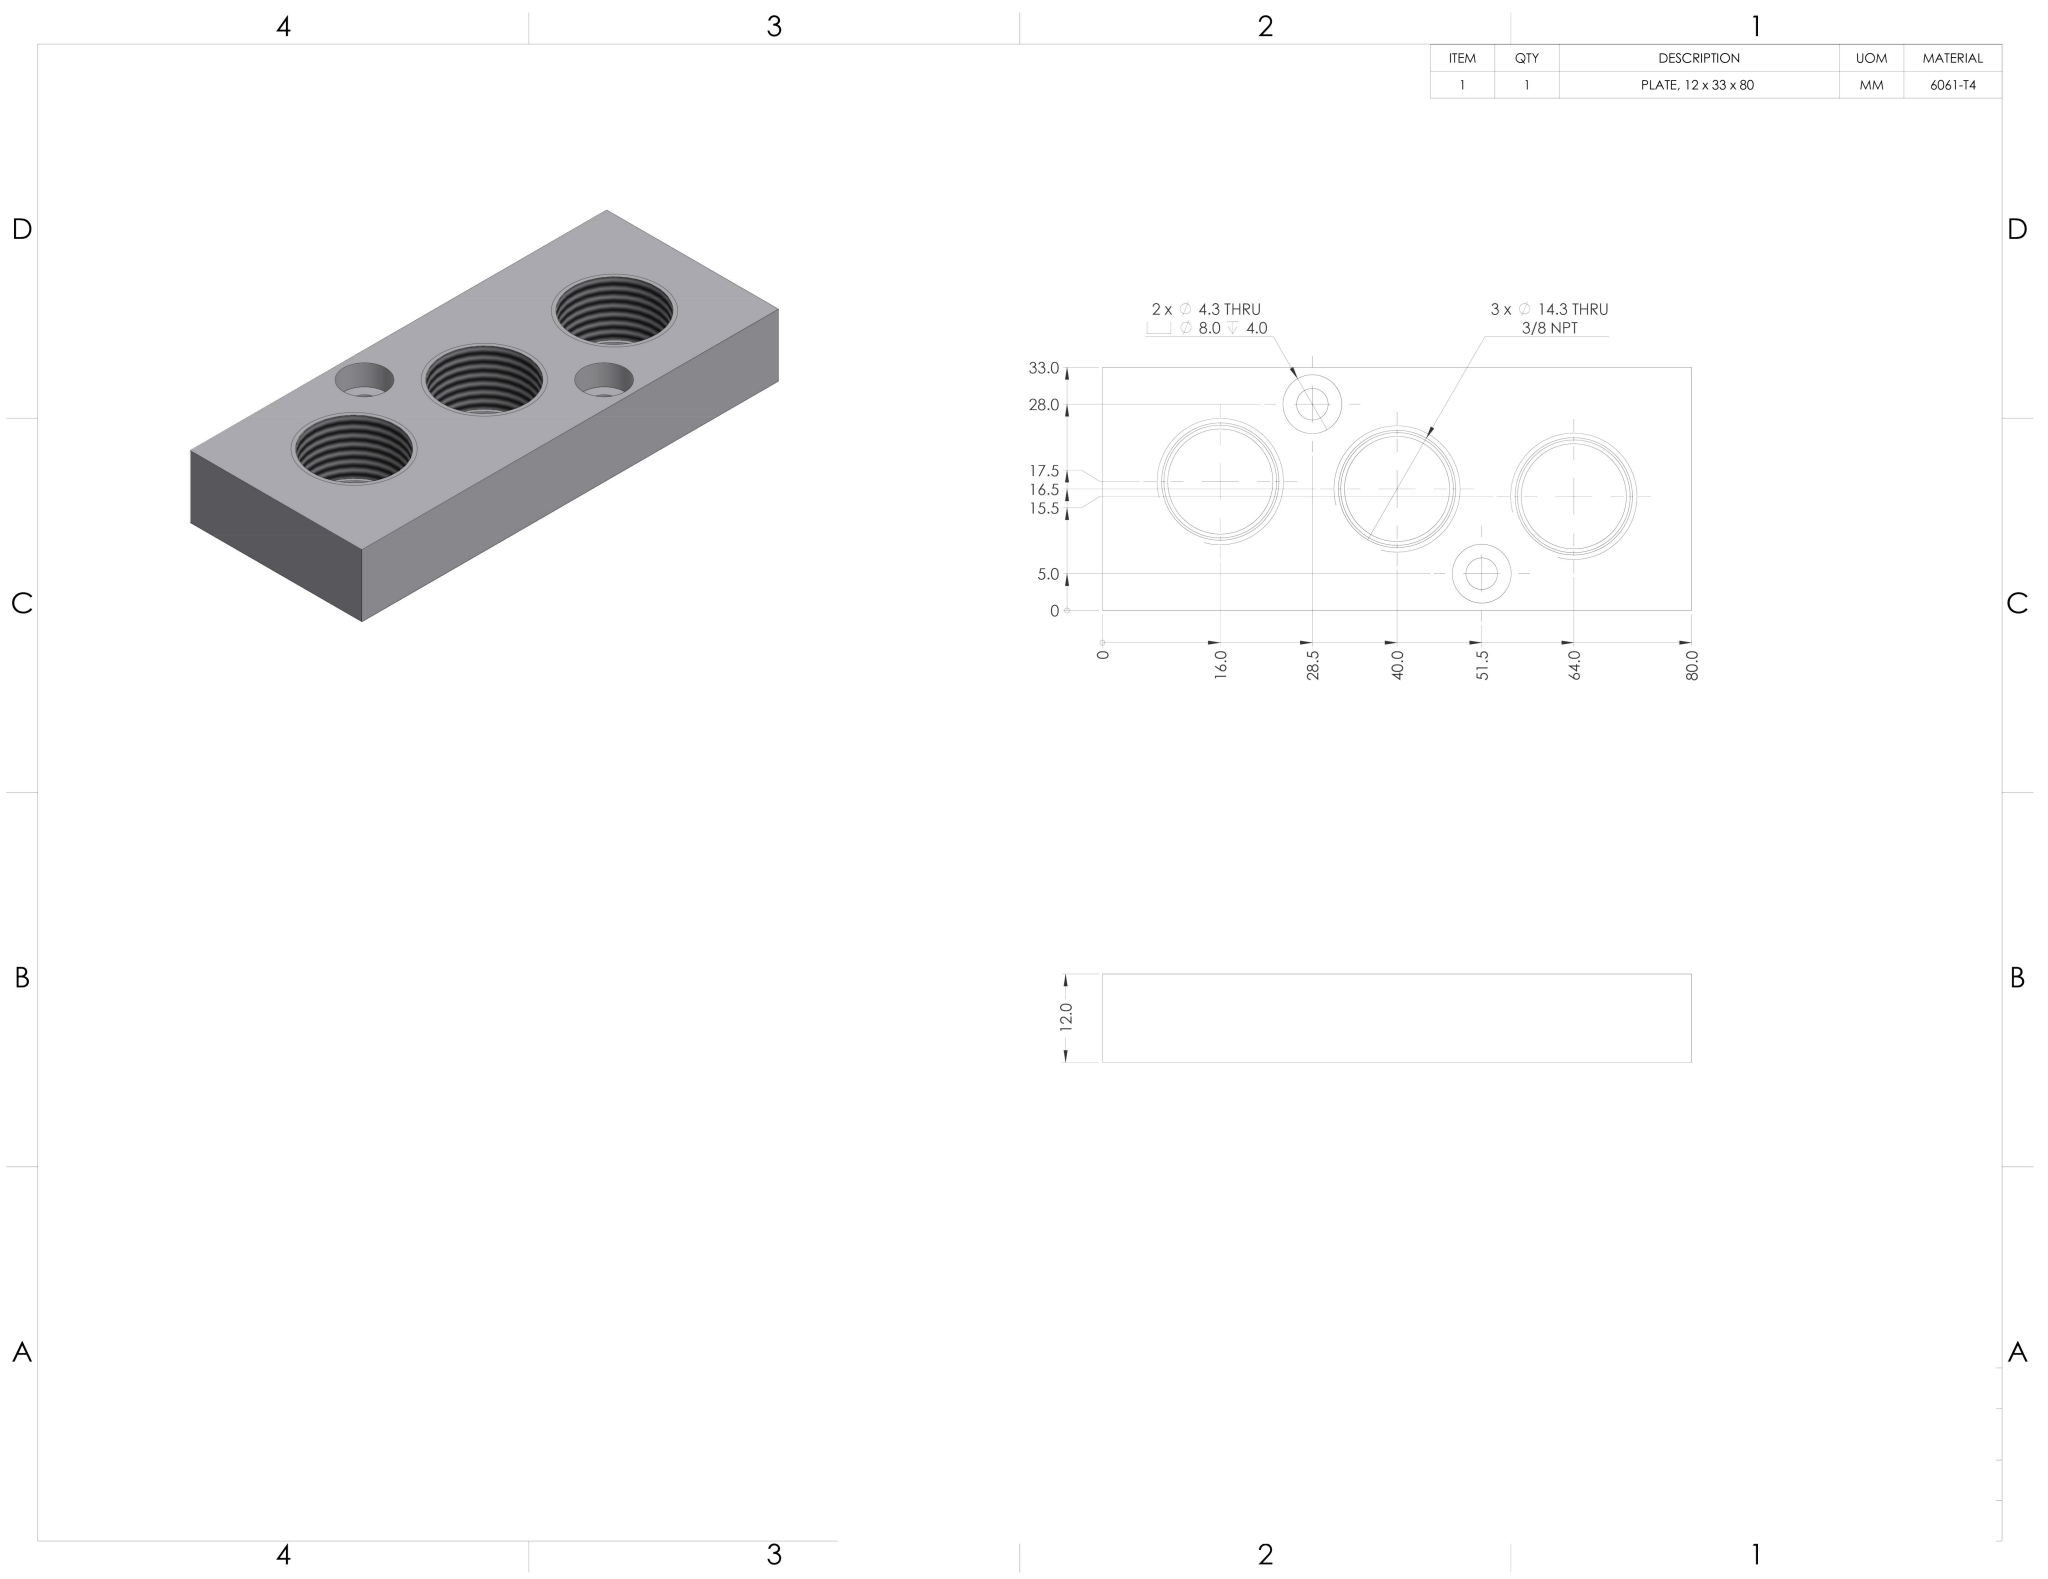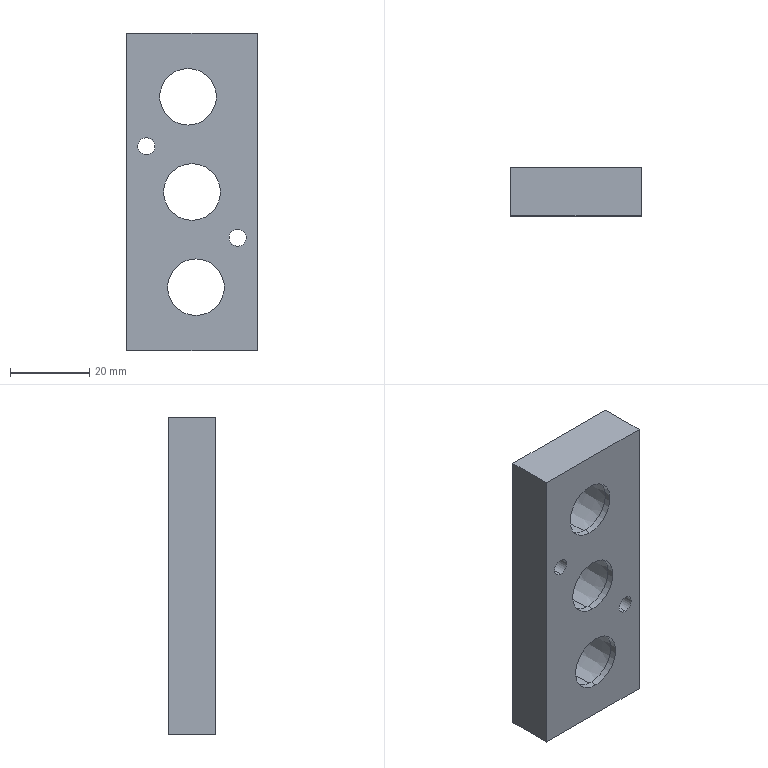Part | NX | mm | 1 solid | 31 faces | box 33 x 12 x 80 mm | volume 24310 mm3 | cylinder 14 | plane 11 | cone 6 | commonest cylinder face diameters 14.275 x6 8 x4 4.3 x4